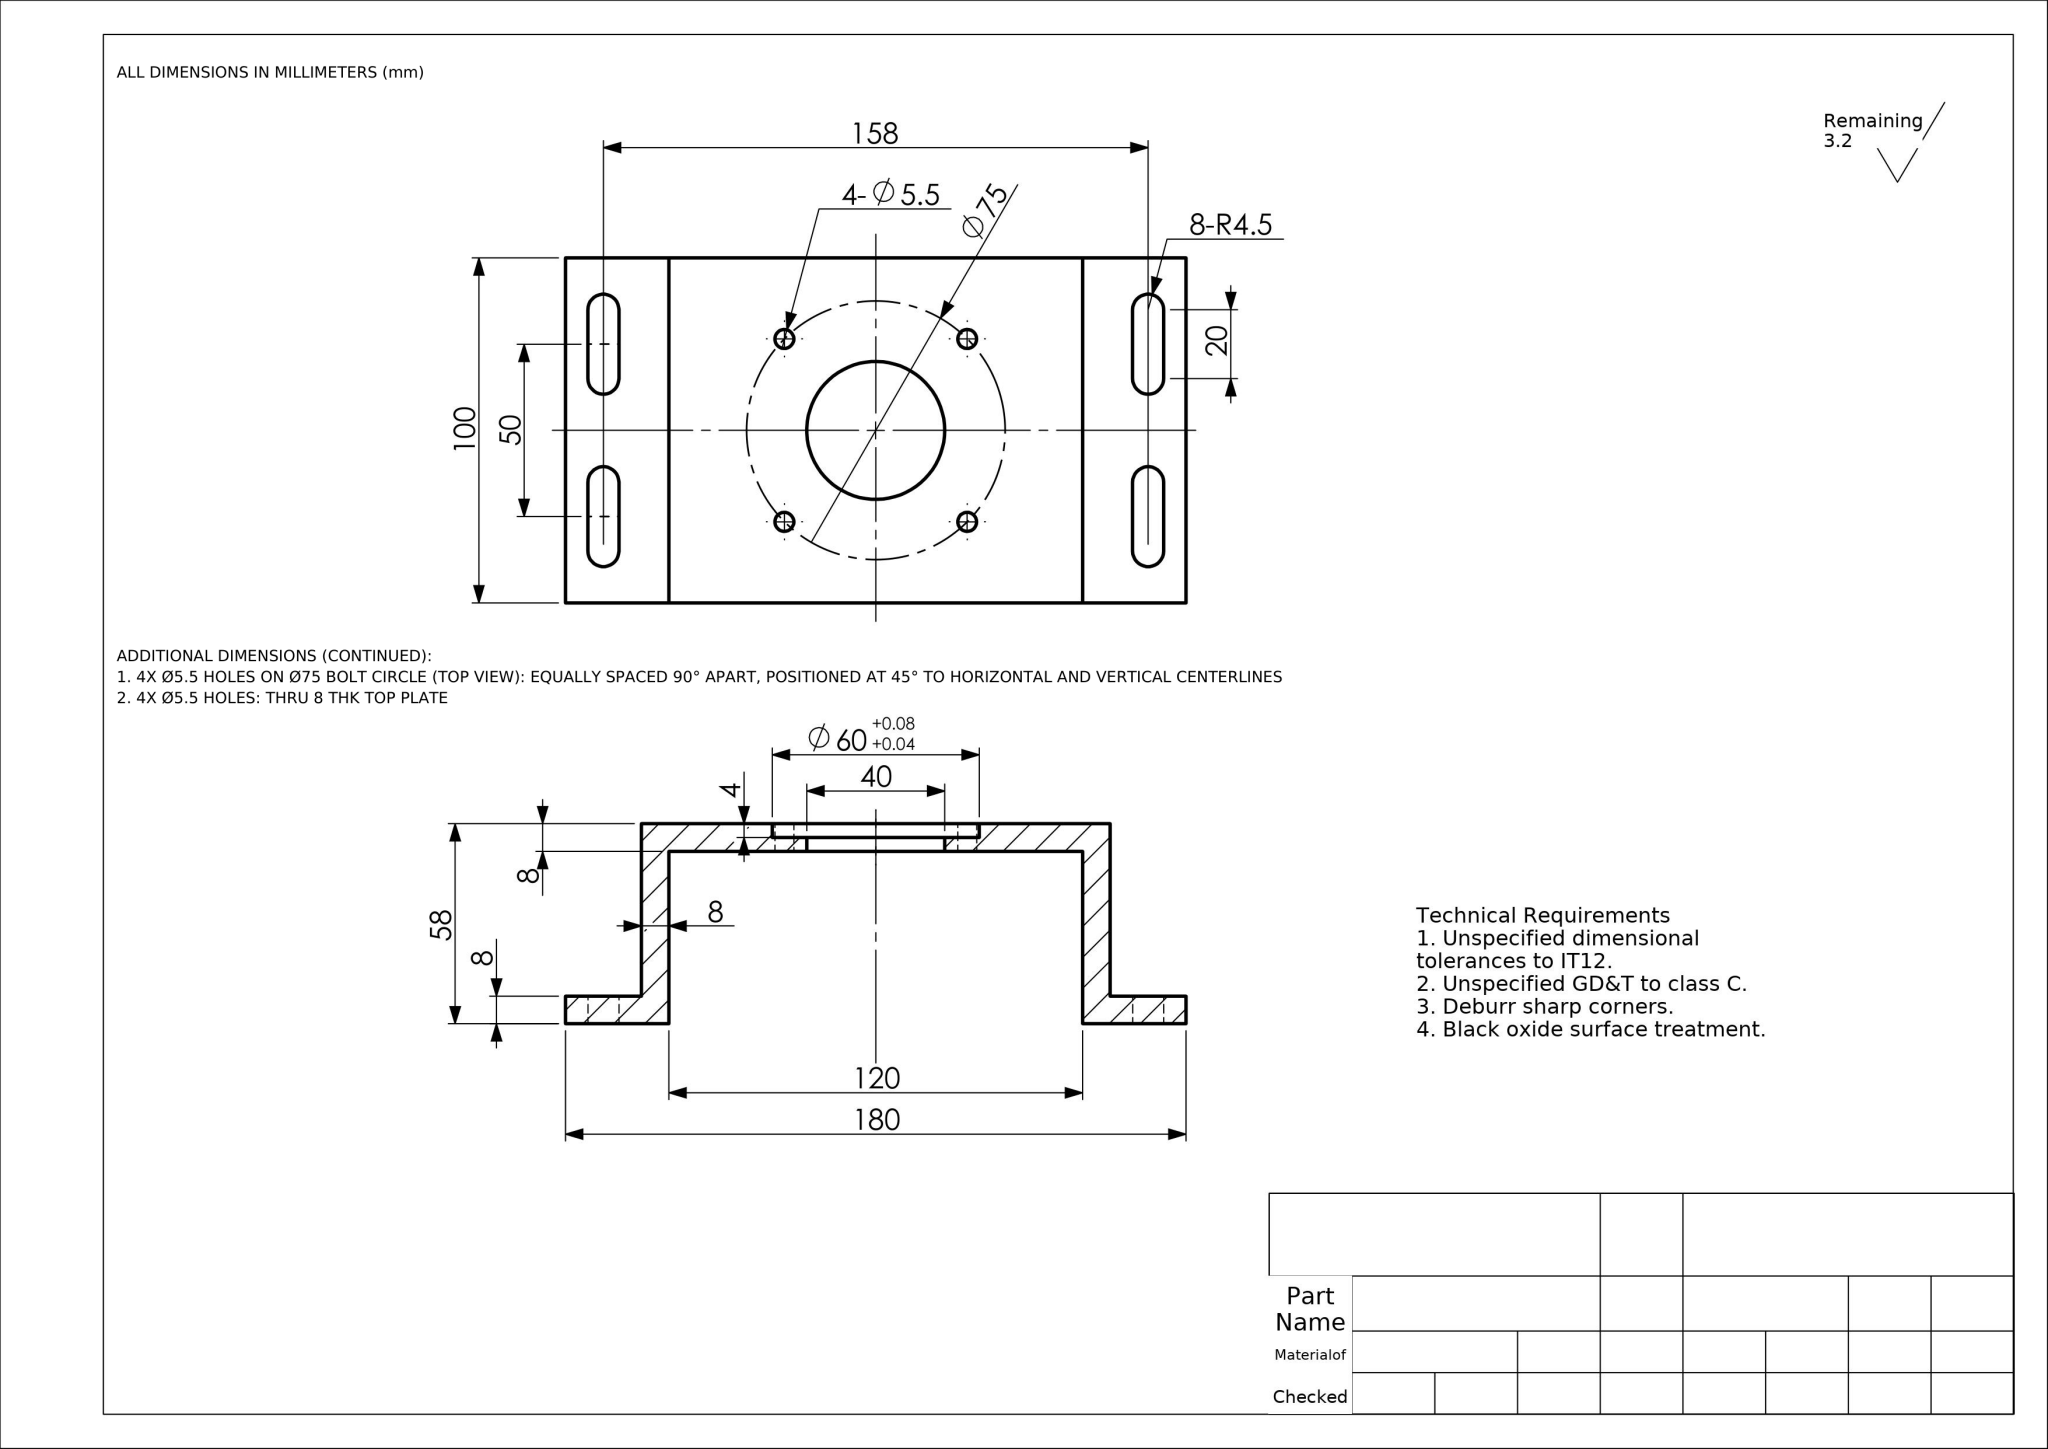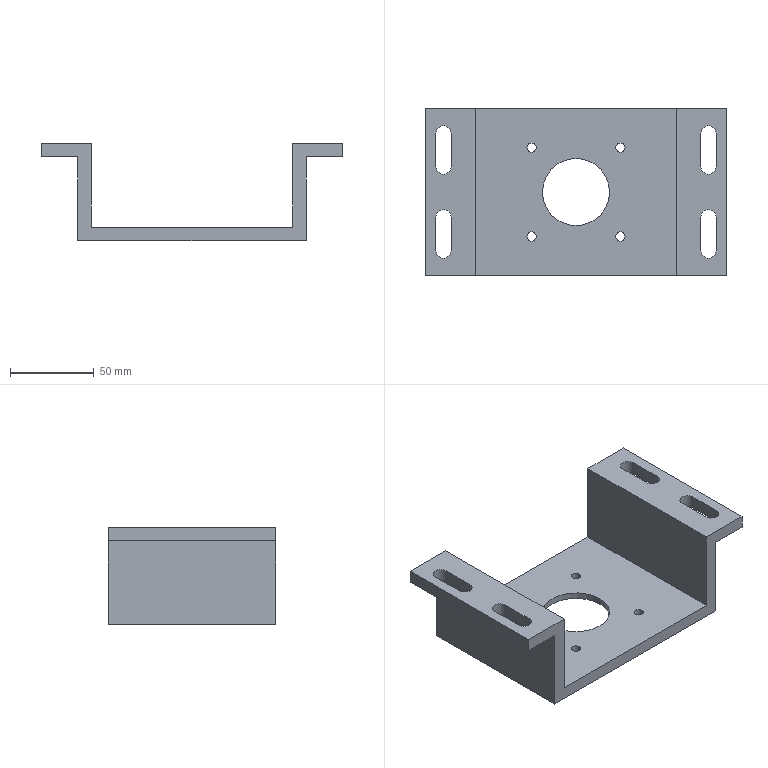Part | NX | mm | 1 solid | 43 faces | box 180 x 100 x 58 mm | volume 199108 mm3 | plane 23 | cylinder 20 | commonest cylinder face diameters 5.5 x8 9 x8 60 x2 40 x2